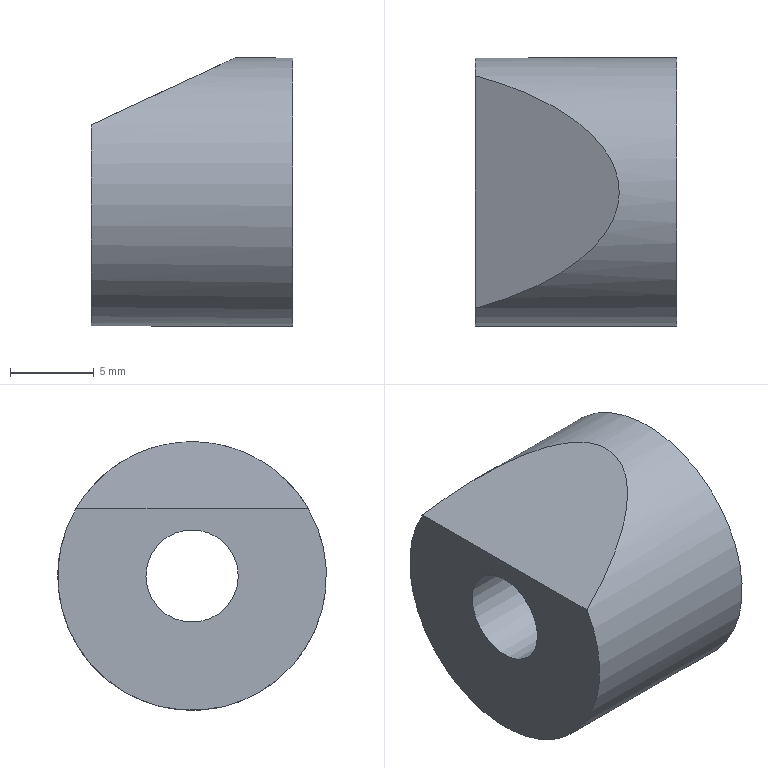Component | NX | LOCKING_SLEEVE | 1 solid | 5 faces | box 12 x 16 x 16 mm | volume 1989 mm3 | plane 3 | cylinder 2 | commonest cylinder face diameters 16 x1 5.5 x1
STEP:
#1=CARTESIAN_POINT('',(0.,0.,0.));
#2=DIRECTION('',(0.,0.,1.));
#3=DIRECTION('',(1.,0.,0.));
#4=AXIS2_PLACEMENT_3D('',#1,#2,#3);
#5=CARTESIAN_POINT('',(90.666,170.327,156.15));
#6=VERTEX_POINT('',#5);
#7=CARTESIAN_POINT('',(90.666,171.398,152.15));
#8=VERTEX_POINT('',#7);
#9=CARTESIAN_POINT('',(90.666,163.398,152.15));
#10=DIRECTION('',(1.,0.,0.));
#11=DIRECTION('',(0.,1.,0.));
#12=AXIS2_PLACEMENT_3D('',#9,#10,#11);
#13=CIRCLE('',#12,8.);
#14=CARTESIAN_POINT('',(90.666,163.398,152.15));
#15=DIRECTION('',(-1.,0.,0.));
#16=DIRECTION('',(0.,0.,1.));
#17=AXIS2_PLACEMENT_3D('',#14,#15,#16);
#18=CYLINDRICAL_SURFACE('',#17,8.);
#19=CARTESIAN_POINT('',(7.854,0.));
#20=DIRECTION('',(-1.,0.));
#21=VECTOR('',#20,1.);
#22=LINE('',#19,#21);
#23=(GEOMETRIC_REPRESENTATION_CONTEXT(2)PARAMETRIC_REPRESENTATION_CONTEXT()REPRESENTATION_CONTEXT('',''));
#24=DEFINITIONAL_REPRESENTATION('',(#22),#23);
#25=PCURVE('',#18,#24);
#26=CARTESIAN_POINT('',(90.666,163.398,152.15));
#27=DIRECTION('',(1.,0.,0.));
#28=DIRECTION('',(0.,0.,-1.));
#29=AXIS2_PLACEMENT_3D('',#26,#27,#28);
#30=PLANE('',#29);
#31=CARTESIAN_POINT('',(0.,0.));
#32=DIRECTION('',(0.,1.));
#33=AXIS2_PLACEMENT_2D('',#31,#32);
#34=CIRCLE('',#33,8.);
#35=(GEOMETRIC_REPRESENTATION_CONTEXT(2)PARAMETRIC_REPRESENTATION_CONTEXT()REPRESENTATION_CONTEXT('',''));
#36=DEFINITIONAL_REPRESENTATION('',(#34),#35);
#37=PCURVE('',#30,#36);
#38=SURFACE_CURVE('',#13,(#25,#37),.PCURVE_S1.);
#39=EDGE_CURVE('',#6,#8,#38,.T.);
#40=ORIENTED_EDGE('',*,*,#39,.F.);
#41=CARTESIAN_POINT('',(78.666,170.327,156.15));
#42=VERTEX_POINT('',#41);
#43=CARTESIAN_POINT('',(90.666,170.327,156.15));
#44=CARTESIAN_POINT('',(78.666,170.327,156.15));
#45=B_SPLINE_CURVE_WITH_KNOTS('',1,(#43,#44),.UNSPECIFIED.,.F.,.F.,(2,2),(0.,12.),.PIECEWISE_BEZIER_KNOTS.);
#46=CARTESIAN_POINT('',(7.33,0.));
#47=DIRECTION('',(0.,1.));
#48=VECTOR('',#47,1.);
#49=LINE('',#46,#48);
#50=(GEOMETRIC_REPRESENTATION_CONTEXT(2)PARAMETRIC_REPRESENTATION_CONTEXT()REPRESENTATION_CONTEXT('',''));
#51=DEFINITIONAL_REPRESENTATION('',(#49),#50);
#52=PCURVE('',#18,#51);
#53=CARTESIAN_POINT('',(1.047,0.));
#54=DIRECTION('',(0.,1.));
#55=VECTOR('',#54,1.);
#56=LINE('',#53,#55);
#57=(GEOMETRIC_REPRESENTATION_CONTEXT(2)PARAMETRIC_REPRESENTATION_CONTEXT()REPRESENTATION_CONTEXT('',''));
#58=DEFINITIONAL_REPRESENTATION('',(#56),#57);
#59=PCURVE('',#18,#58);
#60=SEAM_CURVE('',#45,(#52,#59),.PCURVE_S1.);
#61=EDGE_CURVE('',#6,#42,#60,.T.);
#62=ORIENTED_EDGE('',*,*,#61,.T.);
#63=CARTESIAN_POINT('',(78.666,156.47,156.15));
#64=VERTEX_POINT('',#63);
#65=CARTESIAN_POINT('',(70.088,163.398,152.15));
#66=DIRECTION('',(-0.4226,0.,0.9063));
#67=DIRECTION('',(-0.9063,0.,-0.4226));
#68=AXIS2_PLACEMENT_3D('',#65,#66,#67);
#69=ELLIPSE('',#68,18.93,8.);
#70=CARTESIAN_POINT('',(5.236,12.));
#71=CARTESIAN_POINT('',(5.268,11.528));
#72=CARTESIAN_POINT('',(5.331,10.612));
#73=CARTESIAN_POINT('',(5.426,9.326));
#74=CARTESIAN_POINT('',(5.522,8.143));
#75=CARTESIAN_POINT('',(5.617,7.072));
#76=CARTESIAN_POINT('',(5.712,6.124));
#77=CARTESIAN_POINT('',(5.807,5.306));
#78=CARTESIAN_POINT('',(5.902,4.627));
#79=CARTESIAN_POINT('',(5.998,4.092));
#80=CARTESIAN_POINT('',(6.093,3.707));
#81=CARTESIAN_POINT('',(6.188,3.474));
#82=CARTESIAN_POINT('',(6.283,3.396));
#83=CARTESIAN_POINT('',(6.378,3.474));
#84=CARTESIAN_POINT('',(6.474,3.707));
#85=CARTESIAN_POINT('',(6.569,4.092));
#86=CARTESIAN_POINT('',(6.664,4.627));
#87=CARTESIAN_POINT('',(6.759,5.306));
#88=CARTESIAN_POINT('',(6.854,6.124));
#89=CARTESIAN_POINT('',(6.95,7.072));
#90=CARTESIAN_POINT('',(7.045,8.143));
#91=CARTESIAN_POINT('',(7.14,9.326));
#92=CARTESIAN_POINT('',(7.235,10.612));
#93=CARTESIAN_POINT('',(7.299,11.528));
#94=CARTESIAN_POINT('',(7.33,12.));
#95=B_SPLINE_CURVE_WITH_KNOTS('',3,(#70,#71,#72,#73,#74,#75,#76,#77,#78,#79,#80,#81,#82,#83,#84,#85,#86,#87,#88,#89,#90,#91,#92,#93,#94),.UNSPECIFIED.,.F.,.F.,(4,1,1,1,1,1,1,1,1,1,1,1,1,1,1,1,1,1,1,1,1,1,4),(2.094,2.19,2.285,2.38,2.475,2.57,2.666,2.761,2.856,2.951,3.046,3.142,3.237,3.332,3.427,3.522,3.618,3.713,3.808,3.903,3.998,4.094,4.189),.QUASI_UNIFORM_KNOTS.);
#96=(GEOMETRIC_REPRESENTATION_CONTEXT(2)PARAMETRIC_REPRESENTATION_CONTEXT()REPRESENTATION_CONTEXT('',''));
#97=DEFINITIONAL_REPRESENTATION('',(#95),#96);
#98=PCURVE('',#18,#97);
#99=CARTESIAN_POINT('',(78.666,151.398,156.15));
#100=DIRECTION('',(-0.4226,0.,0.9063));
#101=DIRECTION('',(0.9063,0.,0.4226));
#102=AXIS2_PLACEMENT_3D('',#99,#100,#101);
#103=PLANE('',#102);
#104=CARTESIAN_POINT('',(-9.465,12.));
#105=DIRECTION('',(-1.,0.));
#106=AXIS2_PLACEMENT_2D('',#104,#105);
#107=ELLIPSE('',#106,18.93,8.);
#108=(GEOMETRIC_REPRESENTATION_CONTEXT(2)PARAMETRIC_REPRESENTATION_CONTEXT()REPRESENTATION_CONTEXT('',''));
#109=DEFINITIONAL_REPRESENTATION('',(#107),#108);
#110=PCURVE('',#103,#109);
#111=SURFACE_CURVE('',#69,(#98,#110),.PCURVE_S1.);
#112=EDGE_CURVE('',#64,#42,#111,.T.);
#113=ORIENTED_EDGE('',*,*,#112,.F.);
#114=CARTESIAN_POINT('',(78.666,163.398,152.15));
#115=DIRECTION('',(1.,0.,0.));
#116=DIRECTION('',(0.,1.,0.));
#117=AXIS2_PLACEMENT_3D('',#114,#115,#116);
#118=CIRCLE('',#117,8.);
#119=CARTESIAN_POINT('',(7.854,12.));
#120=DIRECTION('',(-1.,0.));
#121=VECTOR('',#120,1.);
#122=LINE('',#119,#121);
#123=(GEOMETRIC_REPRESENTATION_CONTEXT(2)PARAMETRIC_REPRESENTATION_CONTEXT()REPRESENTATION_CONTEXT('',''));
#124=DEFINITIONAL_REPRESENTATION('',(#122),#123);
#125=PCURVE('',#18,#124);
#126=CARTESIAN_POINT('',(78.666,163.398,152.15));
#127=DIRECTION('',(1.,0.,0.));
#128=DIRECTION('',(0.,0.,-1.));
#129=AXIS2_PLACEMENT_3D('',#126,#127,#128);
#130=PLANE('',#129);
#131=CARTESIAN_POINT('',(0.,0.));
#132=DIRECTION('',(0.,1.));
#133=AXIS2_PLACEMENT_2D('',#131,#132);
#134=CIRCLE('',#133,8.);
#135=(GEOMETRIC_REPRESENTATION_CONTEXT(2)PARAMETRIC_REPRESENTATION_CONTEXT()REPRESENTATION_CONTEXT('',''));
#136=DEFINITIONAL_REPRESENTATION('',(#134),#135);
#137=PCURVE('',#130,#136);
#138=SURFACE_CURVE('',#118,(#125,#137),.PCURVE_S1.);
#139=EDGE_CURVE('',#64,#42,#138,.T.);
#140=ORIENTED_EDGE('',*,*,#139,.T.);
#141=ORIENTED_EDGE('',*,*,#61,.F.);
#142=CARTESIAN_POINT('',(90.666,163.398,152.15));
#143=DIRECTION('',(1.,0.,0.));
#144=DIRECTION('',(0.,1.,0.));
#145=AXIS2_PLACEMENT_3D('',#142,#143,#144);
#146=CIRCLE('',#145,8.);
#147=CARTESIAN_POINT('',(1.571,0.));
#148=DIRECTION('',(-1.,0.));
#149=VECTOR('',#148,1.);
#150=LINE('',#147,#149);
#151=(GEOMETRIC_REPRESENTATION_CONTEXT(2)PARAMETRIC_REPRESENTATION_CONTEXT()REPRESENTATION_CONTEXT('',''));
#152=DEFINITIONAL_REPRESENTATION('',(#150),#151);
#153=PCURVE('',#18,#152);
#154=CARTESIAN_POINT('',(0.,0.));
#155=DIRECTION('',(0.,1.));
#156=AXIS2_PLACEMENT_2D('',#154,#155);
#157=CIRCLE('',#156,8.);
#158=(GEOMETRIC_REPRESENTATION_CONTEXT(2)PARAMETRIC_REPRESENTATION_CONTEXT()REPRESENTATION_CONTEXT('',''));
#159=DEFINITIONAL_REPRESENTATION('',(#157),#158);
#160=PCURVE('',#30,#159);
#161=SURFACE_CURVE('',#146,(#153,#160),.PCURVE_S1.);
#162=EDGE_CURVE('',#8,#6,#161,.T.);
#163=ORIENTED_EDGE('',*,*,#162,.F.);
#164=EDGE_LOOP('',(#40,#62,#113,#140,#141,#163));
#165=FACE_BOUND('',#164,.T.);
#166=ADVANCED_FACE('',(#165),#18,.T.);
#167=CARTESIAN_POINT('',(90.666,166.148,152.15));
#168=VERTEX_POINT('',#167);
#169=CARTESIAN_POINT('',(90.666,163.398,152.15));
#170=DIRECTION('',(1.,0.,0.));
#171=DIRECTION('',(0.,1.,0.));
#172=AXIS2_PLACEMENT_3D('',#169,#170,#171);
#173=CIRCLE('',#172,2.75);
#174=CARTESIAN_POINT('',(0.,0.));
#175=DIRECTION('',(0.,1.));
#176=AXIS2_PLACEMENT_2D('',#174,#175);
#177=CIRCLE('',#176,2.75);
#178=(GEOMETRIC_REPRESENTATION_CONTEXT(2)PARAMETRIC_REPRESENTATION_CONTEXT()REPRESENTATION_CONTEXT('',''));
#179=DEFINITIONAL_REPRESENTATION('',(#177),#178);
#180=PCURVE('',#30,#179);
#181=CARTESIAN_POINT('',(78.666,163.398,152.15));
#182=DIRECTION('',(1.,0.,0.));
#183=DIRECTION('',(0.,0.,-1.));
#184=AXIS2_PLACEMENT_3D('',#181,#182,#183);
#185=CYLINDRICAL_SURFACE('',#184,2.75);
#186=CARTESIAN_POINT('',(1.571,12.));
#187=DIRECTION('',(1.,0.));
#188=VECTOR('',#187,1.);
#189=LINE('',#186,#188);
#190=(GEOMETRIC_REPRESENTATION_CONTEXT(2)PARAMETRIC_REPRESENTATION_CONTEXT()REPRESENTATION_CONTEXT('',''));
#191=DEFINITIONAL_REPRESENTATION('',(#189),#190);
#192=PCURVE('',#185,#191);
#193=SURFACE_CURVE('',#173,(#180,#192),.PCURVE_S1.);
#194=EDGE_CURVE('',#168,#168,#193,.T.);
#195=ORIENTED_EDGE('',*,*,#194,.F.);
#196=EDGE_LOOP('',(#195));
#197=FACE_BOUND('',#196,.T.);
#198=ORIENTED_EDGE('',*,*,#162,.T.);
#199=ORIENTED_EDGE('',*,*,#39,.T.);
#200=EDGE_LOOP('',(#198,#199));
#201=FACE_BOUND('',#200,.T.);
#202=ADVANCED_FACE('',(#197,#201),#30,.T.);
#203=CARTESIAN_POINT('',(78.666,166.148,152.15));
#204=VERTEX_POINT('',#203);
#205=CARTESIAN_POINT('',(78.666,163.398,152.15));
#206=DIRECTION('',(-1.,0.,0.));
#207=DIRECTION('',(0.,1.,0.));
#208=AXIS2_PLACEMENT_3D('',#205,#206,#207);
#209=CIRCLE('',#208,2.75);
#210=CARTESIAN_POINT('',(0.,2.75));
#211=CARTESIAN_POINT('',(4.763,2.75));
#212=CARTESIAN_POINT('',(2.382,-1.375));
#213=CARTESIAN_POINT('',(0.,-5.5));
#214=CARTESIAN_POINT('',(-2.382,-1.375));
#215=CARTESIAN_POINT('',(-4.763,2.75));
#216=CARTESIAN_POINT('',(0.,2.75));
#217=(BOUNDED_CURVE()B_SPLINE_CURVE(2,(#210,#211,#212,#213,#214,#215,#216),.UNSPECIFIED.,.T.,.F.)B_SPLINE_CURVE_WITH_KNOTS((1,2,2,2,2,1),(-2.094,0.,2.094,4.189,6.283,8.378),.UNSPECIFIED.)CURVE()GEOMETRIC_REPRESENTATION_ITEM()RATIONAL_B_SPLINE_CURVE((1.,0.5,1.,0.5,1.,0.5,1.))REPRESENTATION_ITEM(''));
#218=(GEOMETRIC_REPRESENTATION_CONTEXT(2)PARAMETRIC_REPRESENTATION_CONTEXT()REPRESENTATION_CONTEXT('',''));
#219=DEFINITIONAL_REPRESENTATION('',(#217),#218);
#220=PCURVE('',#130,#219);
#221=CARTESIAN_POINT('',(7.854,0.));
#222=DIRECTION('',(-1.,0.));
#223=VECTOR('',#222,1.);
#224=LINE('',#221,#223);
#225=(GEOMETRIC_REPRESENTATION_CONTEXT(2)PARAMETRIC_REPRESENTATION_CONTEXT()REPRESENTATION_CONTEXT('',''));
#226=DEFINITIONAL_REPRESENTATION('',(#224),#225);
#227=PCURVE('',#185,#226);
#228=SURFACE_CURVE('',#209,(#220,#227),.PCURVE_S1.);
#229=EDGE_CURVE('',#204,#204,#228,.T.);
#230=ORIENTED_EDGE('',*,*,#229,.F.);
#231=EDGE_LOOP('',(#230));
#232=FACE_BOUND('',#231,.T.);
#233=ORIENTED_EDGE('',*,*,#139,.F.);
#234=CARTESIAN_POINT('',(78.666,151.398,156.15));
#235=DIRECTION('',(0.,-1.,0.));
#236=VECTOR('',#235,1.);
#237=LINE('',#234,#236);
#238=CARTESIAN_POINT('',(-4.,-12.));
#239=DIRECTION('',(0.,-1.));
#240=VECTOR('',#239,1.);
#241=LINE('',#238,#240);
#242=(GEOMETRIC_REPRESENTATION_CONTEXT(2)PARAMETRIC_REPRESENTATION_CONTEXT()REPRESENTATION_CONTEXT('',''));
#243=DEFINITIONAL_REPRESENTATION('',(#241),#242);
#244=PCURVE('',#130,#243);
#245=CARTESIAN_POINT('',(0.,0.));
#246=DIRECTION('',(0.,-1.));
#247=VECTOR('',#246,1.);
#248=LINE('',#245,#247);
#249=(GEOMETRIC_REPRESENTATION_CONTEXT(2)PARAMETRIC_REPRESENTATION_CONTEXT()REPRESENTATION_CONTEXT('',''));
#250=DEFINITIONAL_REPRESENTATION('',(#248),#249);
#251=PCURVE('',#103,#250);
#252=SURFACE_CURVE('',#237,(#244,#251),.PCURVE_S1.);
#253=EDGE_CURVE('',#42,#64,#252,.T.);
#254=ORIENTED_EDGE('',*,*,#253,.F.);
#255=EDGE_LOOP('',(#233,#254));
#256=FACE_BOUND('',#255,.T.);
#257=ADVANCED_FACE('',(#232,#256),#130,.F.);
#258=ORIENTED_EDGE('',*,*,#229,.F.);
#259=CARTESIAN_POINT('',(78.666,166.148,152.15));
#260=CARTESIAN_POINT('',(90.666,166.148,152.15));
#261=B_SPLINE_CURVE_WITH_KNOTS('',1,(#259,#260),.UNSPECIFIED.,.F.,.F.,(2,2),(0.,12.),.PIECEWISE_BEZIER_KNOTS.);
#262=CARTESIAN_POINT('',(7.854,0.));
#263=DIRECTION('',(0.,1.));
#264=VECTOR('',#263,1.);
#265=LINE('',#262,#264);
#266=(GEOMETRIC_REPRESENTATION_CONTEXT(2)PARAMETRIC_REPRESENTATION_CONTEXT()REPRESENTATION_CONTEXT('',''));
#267=DEFINITIONAL_REPRESENTATION('',(#265),#266);
#268=PCURVE('',#185,#267);
#269=CARTESIAN_POINT('',(1.571,0.));
#270=DIRECTION('',(0.,1.));
#271=VECTOR('',#270,1.);
#272=LINE('',#269,#271);
#273=(GEOMETRIC_REPRESENTATION_CONTEXT(2)PARAMETRIC_REPRESENTATION_CONTEXT()REPRESENTATION_CONTEXT('',''));
#274=DEFINITIONAL_REPRESENTATION('',(#272),#273);
#275=PCURVE('',#185,#274);
#276=SEAM_CURVE('',#261,(#268,#275),.PCURVE_S1.);
#277=EDGE_CURVE('',#204,#168,#276,.T.);
#278=ORIENTED_EDGE('',*,*,#277,.T.);
#279=ORIENTED_EDGE('',*,*,#194,.F.);
#280=ORIENTED_EDGE('',*,*,#277,.F.);
#281=EDGE_LOOP('',(#258,#278,#279,#280));
#282=FACE_BOUND('',#281,.F.);
#283=ADVANCED_FACE('',(#282),#185,.F.);
#284=ORIENTED_EDGE('',*,*,#112,.T.);
#285=ORIENTED_EDGE('',*,*,#253,.T.);
#286=EDGE_LOOP('',(#284,#285));
#287=FACE_BOUND('',#286,.T.);
#288=ADVANCED_FACE('',(#287),#103,.T.);
#289=CLOSED_SHELL('',(#166,#202,#257,#283,#288));
#290=MANIFOLD_SOLID_BREP('',#289);
#291=(LENGTH_UNIT()NAMED_UNIT(*)SI_UNIT(.MILLI.,.METRE.));
#292=UNCERTAINTY_MEASURE_WITH_UNIT(LENGTH_MEASURE(0.000005),#291,'','');
#293=(NAMED_UNIT(*)PLANE_ANGLE_UNIT()SI_UNIT($,.RADIAN.));
#294=(NAMED_UNIT(*)SI_UNIT($,.STERADIAN.)SOLID_ANGLE_UNIT());
#295=(GEOMETRIC_REPRESENTATION_CONTEXT(3)GLOBAL_UNCERTAINTY_ASSIGNED_CONTEXT((#292))GLOBAL_UNIT_ASSIGNED_CONTEXT((#291,#293,#294))REPRESENTATION_CONTEXT('',''));
#296=ADVANCED_BREP_SHAPE_REPRESENTATION('',(#4,#290),#295);